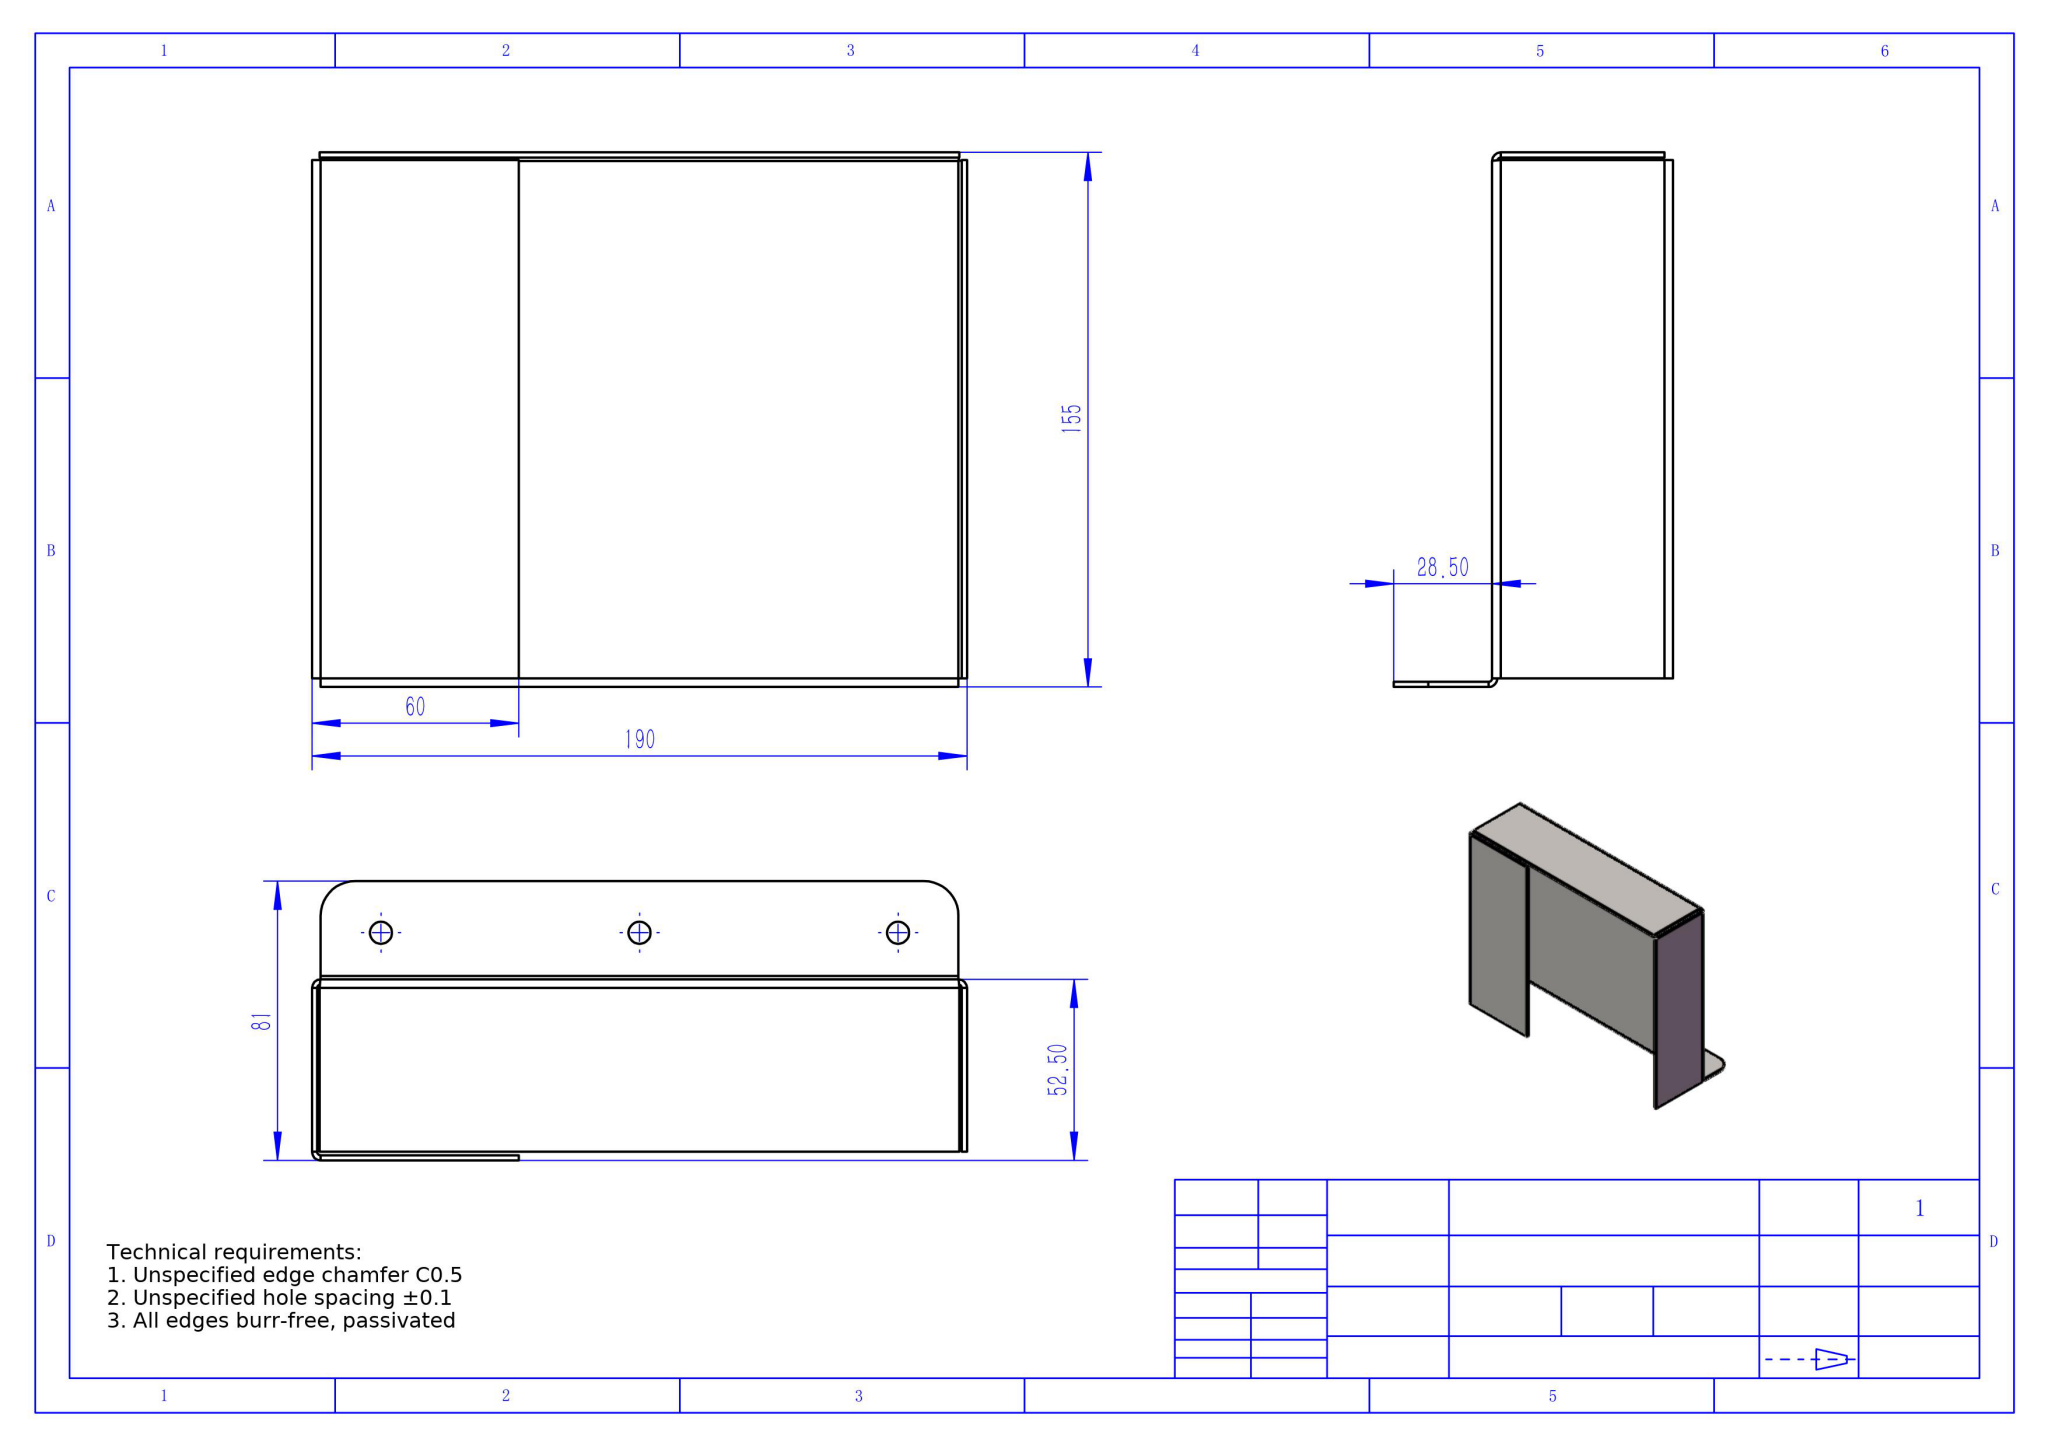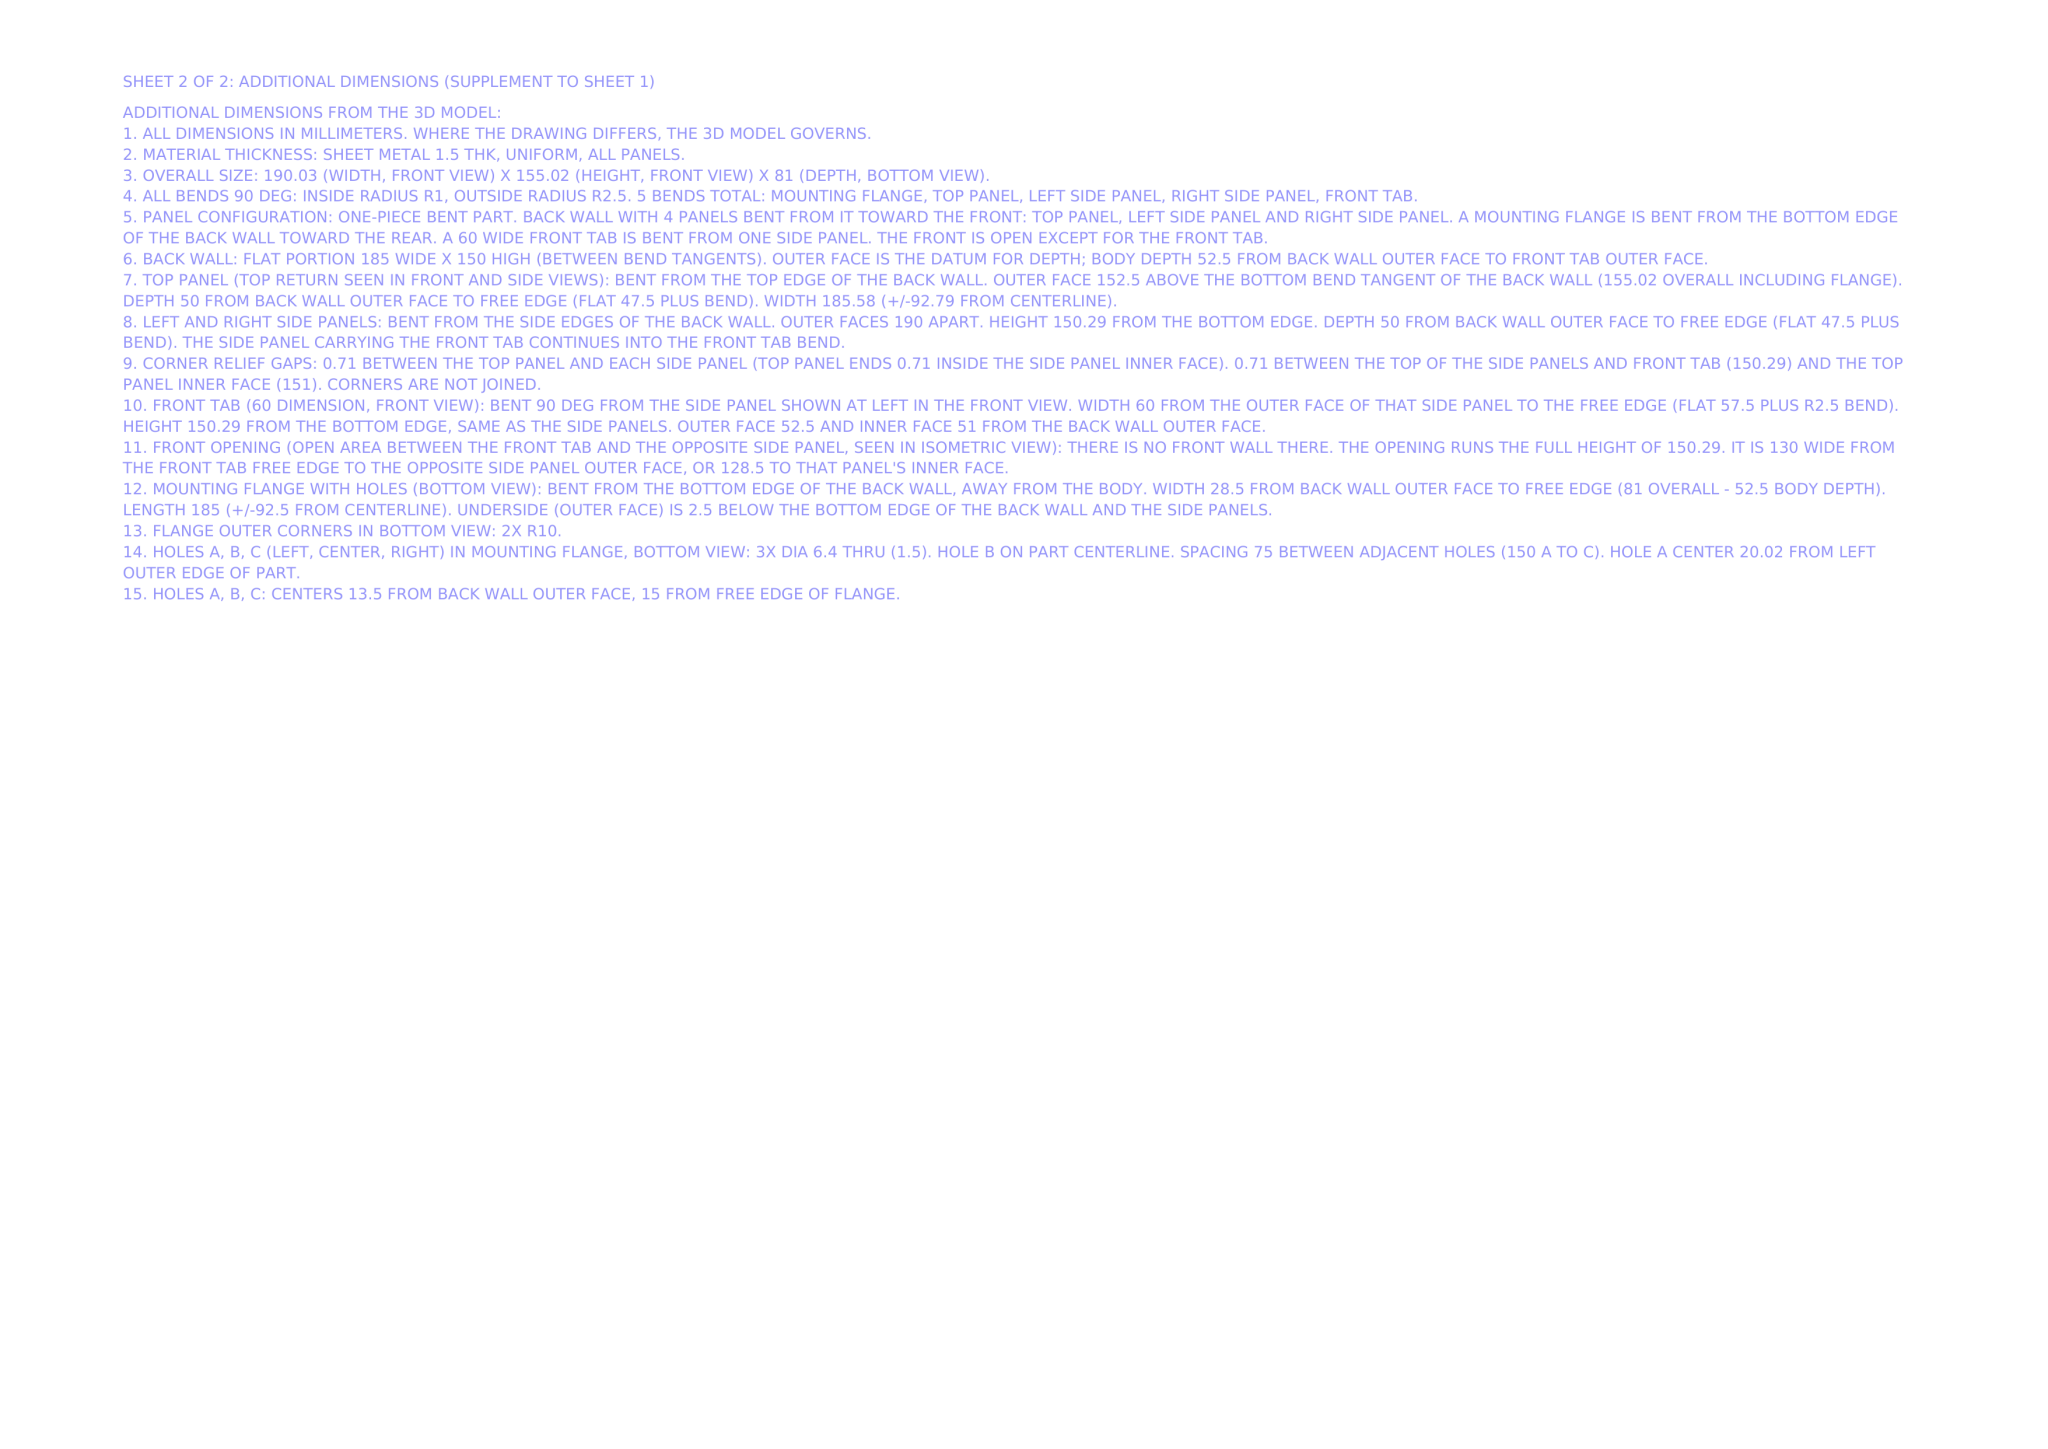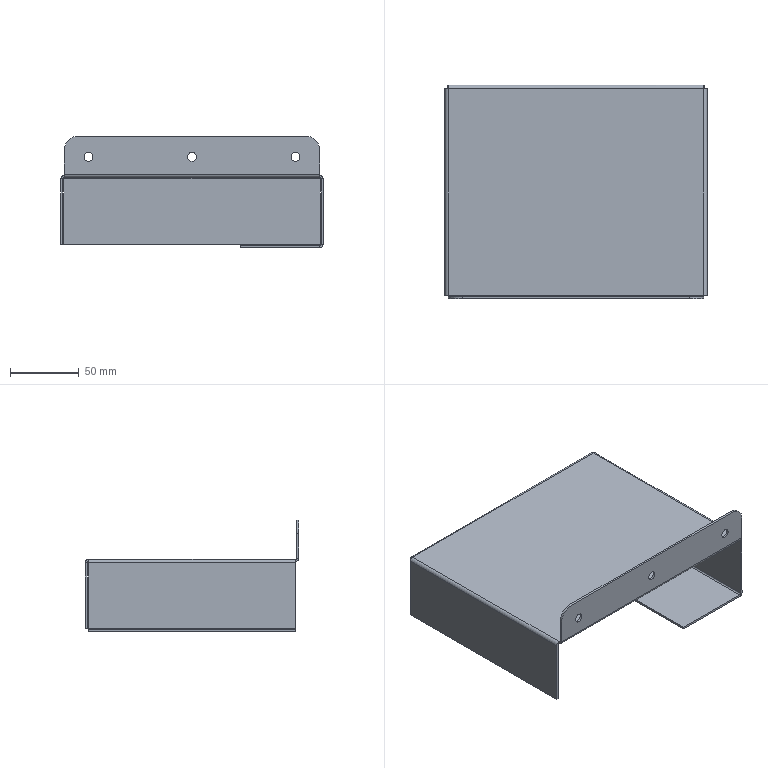Part | NX | mm | 1 solid | 54 faces | box 190 x 155 x 81 mm | volume 100034 mm3 | plane 32 | cylinder 18 | spline 4 | commonest cylinder face diameters 6.4 x6 5 x5 2 x5 20 x2